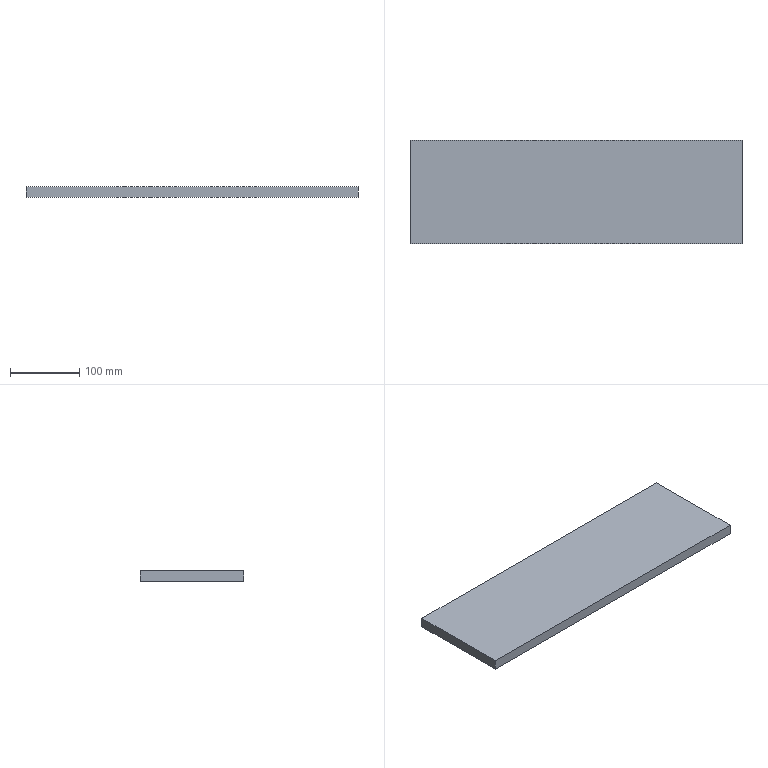Component | SolidWorks | SlidingSupport1122-1 | 1 solid | 6 faces | box 480 x 150 x 15 mm | volume 1080000 mm3 | plane 6
build123d program:
from build123d import *

# Parameters (mm, degrees)
SKETCH1_W           = 480
SKETCH1_H           = 150
BOSS_EXTRUDE1_DEPTH = 15


with BuildPart() as part:
    # Sketch1 → Boss-Extrude1 (new body)
    with BuildSketch(Plane.XY):
        Rectangle(SKETCH1_W, SKETCH1_H)
    extrude(amount=BOSS_EXTRUDE1_DEPTH)


solid = part.part

# Placed as in the assembly
solid = solid.moved(Location((-84.479, -49.348, 874.07), (0, 0, 0)))
STEP:
#1=CARTESIAN_POINT('',(6.123,-4.896,34.412));
#2=VERTEX_POINT('',#1);
#3=CARTESIAN_POINT('',(6.123,1.01,34.412));
#4=VERTEX_POINT('',#3);
#5=CARTESIAN_POINT('',(6.123,-4.896,34.412));
#6=DIRECTION('',(0.,1.,0.));
#7=VECTOR('',#6,39.37);
#8=LINE('',#5,#7);
#9=EDGE_CURVE('',#2,#4,#8,.T.);
#10=ORIENTED_EDGE('',*,*,#9,.T.);
#11=CARTESIAN_POINT('',(6.123,1.01,35.003));
#12=VERTEX_POINT('',#11);
#13=CARTESIAN_POINT('',(6.123,1.01,35.003));
#14=DIRECTION('',(0.,0.,-1.));
#15=VECTOR('',#14,39.37);
#16=LINE('',#13,#15);
#17=EDGE_CURVE('',#12,#4,#16,.T.);
#18=ORIENTED_EDGE('',*,*,#17,.F.);
#19=CARTESIAN_POINT('',(6.123,-4.896,35.003));
#20=VERTEX_POINT('',#19);
#21=CARTESIAN_POINT('',(6.123,-4.896,35.003));
#22=DIRECTION('',(0.,1.,0.));
#23=VECTOR('',#22,39.37);
#24=LINE('',#21,#23);
#25=EDGE_CURVE('',#20,#12,#24,.T.);
#26=ORIENTED_EDGE('',*,*,#25,.F.);
#27=CARTESIAN_POINT('',(6.123,-4.896,35.003));
#28=DIRECTION('',(0.,0.,-1.));
#29=VECTOR('',#28,39.37);
#30=LINE('',#27,#29);
#31=EDGE_CURVE('',#20,#2,#30,.T.);
#32=ORIENTED_EDGE('',*,*,#31,.T.);
#33=EDGE_LOOP('',(#10,#18,#26,#32));
#34=FACE_OUTER_BOUND('',#33,.T.);
#35=CARTESIAN_POINT('',(6.123,-4.896,35.003));
#36=DIRECTION('',(-1.,0.,0.));
#37=DIRECTION('',(0.,0.,1.));
#38=AXIS2_PLACEMENT_3D('',#35,#36,#37);
#39=PLANE('',#38);
#40=ADVANCED_FACE('',(#34),#39,.F.);
#41=CARTESIAN_POINT('',(-12.775,1.01,34.412));
#42=VERTEX_POINT('',#41);
#43=CARTESIAN_POINT('',(-12.775,1.01,34.412));
#44=DIRECTION('',(-1.,0.,0.));
#45=VECTOR('',#44,39.37);
#46=LINE('',#43,#45);
#47=EDGE_CURVE('',#4,#42,#46,.T.);
#48=ORIENTED_EDGE('',*,*,#47,.T.);
#49=CARTESIAN_POINT('',(-12.775,1.01,35.003));
#50=VERTEX_POINT('',#49);
#51=CARTESIAN_POINT('',(-12.775,1.01,35.003));
#52=DIRECTION('',(0.,0.,-1.));
#53=VECTOR('',#52,39.37);
#54=LINE('',#51,#53);
#55=EDGE_CURVE('',#50,#42,#54,.T.);
#56=ORIENTED_EDGE('',*,*,#55,.F.);
#57=CARTESIAN_POINT('',(-12.775,1.01,35.003));
#58=DIRECTION('',(-1.,0.,0.));
#59=VECTOR('',#58,39.37);
#60=LINE('',#57,#59);
#61=EDGE_CURVE('',#12,#50,#60,.T.);
#62=ORIENTED_EDGE('',*,*,#61,.F.);
#63=ORIENTED_EDGE('',*,*,#17,.T.);
#64=EDGE_LOOP('',(#48,#56,#62,#63));
#65=FACE_OUTER_BOUND('',#64,.T.);
#66=CARTESIAN_POINT('',(-12.775,1.01,35.003));
#67=DIRECTION('',(0.,-1.,0.));
#68=DIRECTION('',(0.,0.,-1.));
#69=AXIS2_PLACEMENT_3D('',#66,#67,#68);
#70=PLANE('',#69);
#71=ADVANCED_FACE('',(#65),#70,.F.);
#72=CARTESIAN_POINT('',(-12.775,-4.896,34.412));
#73=VERTEX_POINT('',#72);
#74=CARTESIAN_POINT('',(-12.775,-4.896,34.412));
#75=DIRECTION('',(0.,-1.,0.));
#76=VECTOR('',#75,39.37);
#77=LINE('',#74,#76);
#78=EDGE_CURVE('',#42,#73,#77,.T.);
#79=ORIENTED_EDGE('',*,*,#78,.T.);
#80=CARTESIAN_POINT('',(-12.775,-4.896,35.003));
#81=VERTEX_POINT('',#80);
#82=CARTESIAN_POINT('',(-12.775,-4.896,35.003));
#83=DIRECTION('',(0.,0.,-1.));
#84=VECTOR('',#83,39.37);
#85=LINE('',#82,#84);
#86=EDGE_CURVE('',#81,#73,#85,.T.);
#87=ORIENTED_EDGE('',*,*,#86,.F.);
#88=CARTESIAN_POINT('',(-12.775,-4.896,35.003));
#89=DIRECTION('',(0.,-1.,0.));
#90=VECTOR('',#89,39.37);
#91=LINE('',#88,#90);
#92=EDGE_CURVE('',#50,#81,#91,.T.);
#93=ORIENTED_EDGE('',*,*,#92,.F.);
#94=ORIENTED_EDGE('',*,*,#55,.T.);
#95=EDGE_LOOP('',(#79,#87,#93,#94));
#96=FACE_OUTER_BOUND('',#95,.T.);
#97=CARTESIAN_POINT('',(-12.775,-4.896,35.003));
#98=DIRECTION('',(1.,0.,0.));
#99=DIRECTION('',(0.,0.,-1.));
#100=AXIS2_PLACEMENT_3D('',#97,#98,#99);
#101=PLANE('',#100);
#102=ADVANCED_FACE('',(#96),#101,.F.);
#103=CARTESIAN_POINT('',(-12.775,-4.896,34.412));
#104=DIRECTION('',(1.,0.,0.));
#105=VECTOR('',#104,39.37);
#106=LINE('',#103,#105);
#107=EDGE_CURVE('',#73,#2,#106,.T.);
#108=ORIENTED_EDGE('',*,*,#107,.T.);
#109=ORIENTED_EDGE('',*,*,#31,.F.);
#110=CARTESIAN_POINT('',(-12.775,-4.896,35.003));
#111=DIRECTION('',(1.,0.,0.));
#112=VECTOR('',#111,39.37);
#113=LINE('',#110,#112);
#114=EDGE_CURVE('',#81,#20,#113,.T.);
#115=ORIENTED_EDGE('',*,*,#114,.F.);
#116=ORIENTED_EDGE('',*,*,#86,.T.);
#117=EDGE_LOOP('',(#108,#109,#115,#116));
#118=FACE_OUTER_BOUND('',#117,.T.);
#119=CARTESIAN_POINT('',(-12.775,-4.896,35.003));
#120=DIRECTION('',(0.,1.,0.));
#121=DIRECTION('',(0.,0.,1.));
#122=AXIS2_PLACEMENT_3D('',#119,#120,#121);
#123=PLANE('',#122);
#124=ADVANCED_FACE('',(#118),#123,.F.);
#125=ORIENTED_EDGE('',*,*,#25,.T.);
#126=ORIENTED_EDGE('',*,*,#61,.T.);
#127=ORIENTED_EDGE('',*,*,#92,.T.);
#128=ORIENTED_EDGE('',*,*,#114,.T.);
#129=EDGE_LOOP('',(#125,#126,#127,#128));
#130=FACE_OUTER_BOUND('',#129,.T.);
#131=CARTESIAN_POINT('',(-3.326,-1.943,35.003));
#132=DIRECTION('',(0.,0.,-1.));
#133=DIRECTION('',(-1.,0.,0.));
#134=AXIS2_PLACEMENT_3D('',#131,#132,#133);
#135=PLANE('',#134);
#136=ADVANCED_FACE('',(#130),#135,.F.);
#137=ORIENTED_EDGE('',*,*,#9,.F.);
#138=ORIENTED_EDGE('',*,*,#107,.F.);
#139=ORIENTED_EDGE('',*,*,#78,.F.);
#140=ORIENTED_EDGE('',*,*,#47,.F.);
#141=EDGE_LOOP('',(#137,#138,#139,#140));
#142=FACE_OUTER_BOUND('',#141,.T.);
#143=CARTESIAN_POINT('',(-3.326,-1.943,34.412));
#144=DIRECTION('',(0.,0.,-1.));
#145=DIRECTION('',(-1.,0.,0.));
#146=AXIS2_PLACEMENT_3D('',#143,#144,#145);
#147=PLANE('',#146);
#148=ADVANCED_FACE('',(#142),#147,.T.);
#149=CLOSED_SHELL('',(#40,#71,#102,#124,#136,#148));
#150=MANIFOLD_SOLID_BREP('',#149);
#151=CARTESIAN_POINT('',(0.,0.,0.));
#152=DIRECTION('',(0.,0.,1.));
#153=DIRECTION('',(1.,0.,0.));
#154=AXIS2_PLACEMENT_3D('',#151,#152,#153);
#155=(LENGTH_UNIT()NAMED_UNIT(*)SI_UNIT($,.METRE.));
#156=LENGTH_MEASURE_WITH_UNIT(LENGTH_MEASURE(0.0254),#155);
#157=DIMENSIONAL_EXPONENTS(1.,0.,0.,0.,0.,0.,0.);
#158=(CONVERSION_BASED_UNIT('',#156)LENGTH_UNIT()NAMED_UNIT(#157));
#159=UNCERTAINTY_MEASURE_WITH_UNIT(LENGTH_MEASURE(0.00001),#158,'','');
#160=(NAMED_UNIT(*)PLANE_ANGLE_UNIT()SI_UNIT($,.RADIAN.));
#161=(NAMED_UNIT(*)SI_UNIT($,.STERADIAN.)SOLID_ANGLE_UNIT());
#162=(GEOMETRIC_REPRESENTATION_CONTEXT(3)GLOBAL_UNCERTAINTY_ASSIGNED_CONTEXT((#159))GLOBAL_UNIT_ASSIGNED_CONTEXT((#158,#160,#161))REPRESENTATION_CONTEXT('',''));
#163=ADVANCED_BREP_SHAPE_REPRESENTATION('',(#150,#154),#162);
#164=COLOUR_RGB('',0.7922,0.8196,0.9333);
#165=FILL_AREA_STYLE_COLOUR('',#164);
#166=FILL_AREA_STYLE('',(#165));
#167=SURFACE_STYLE_FILL_AREA(#166);
#168=SURFACE_SIDE_STYLE('',(#167));
#169=SURFACE_STYLE_USAGE(.BOTH.,#168);
#170=PRESENTATION_STYLE_ASSIGNMENT((#169));
#171=STYLED_ITEM('',(#170),#150);
#172=PRESENTATION_LAYER_ASSIGNMENT('','',(#171));
#173=(LENGTH_UNIT()NAMED_UNIT(*)SI_UNIT($,.METRE.));
#174=LENGTH_MEASURE_WITH_UNIT(LENGTH_MEASURE(0.0254),#173);
#175=DIMENSIONAL_EXPONENTS(1.,0.,0.,0.,0.,0.,0.);
#176=(CONVERSION_BASED_UNIT('',#174)LENGTH_UNIT()NAMED_UNIT(#175));
#177=UNCERTAINTY_MEASURE_WITH_UNIT(LENGTH_MEASURE(0.00001),#176,'','');
#178=(NAMED_UNIT(*)PLANE_ANGLE_UNIT()SI_UNIT($,.RADIAN.));
#179=(NAMED_UNIT(*)SI_UNIT($,.STERADIAN.)SOLID_ANGLE_UNIT());
#180=(GEOMETRIC_REPRESENTATION_CONTEXT(3)GLOBAL_UNCERTAINTY_ASSIGNED_CONTEXT((#177))GLOBAL_UNIT_ASSIGNED_CONTEXT((#176,#178,#179))REPRESENTATION_CONTEXT('',''));
#181=MECHANICAL_DESIGN_GEOMETRIC_PRESENTATION_REPRESENTATION('',(#171),#180);